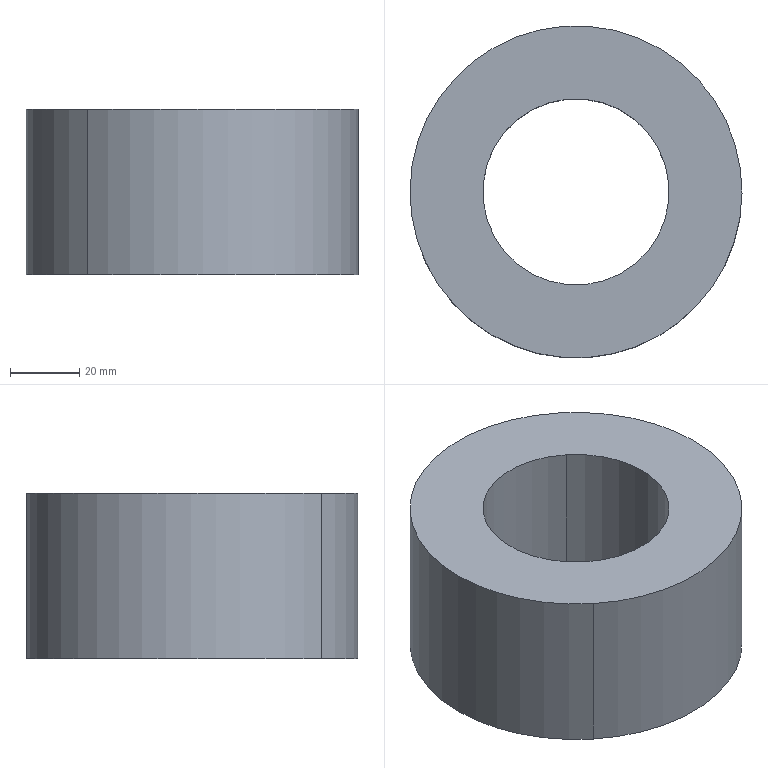Component | SolidWorks | 1-1 | 1 solid | 6 faces | box 96.06 x 96.06 x 48 mm | volume 238346 mm3 | cylinder 4 | plane 2 | commonest cylinder face diameters 53.9 x2 96.06 x2
STEP:
#1=COLOUR_RGB('',0.7922,0.8196,0.9333);
#2=FILL_AREA_STYLE_COLOUR('',#1);
#3=FILL_AREA_STYLE('',(#2));
#4=SURFACE_STYLE_FILL_AREA(#3);
#5=SURFACE_SIDE_STYLE('',(#4));
#6=SURFACE_STYLE_USAGE(.BOTH.,#5);
#7=PRESENTATION_STYLE_ASSIGNMENT((#6));
#8=CARTESIAN_POINT('',(0.6676,0.8247,-1.89));
#9=VERTEX_POINT('',#8);
#10=CARTESIAN_POINT('',(0.6676,0.8247,-3.78));
#11=VERTEX_POINT('',#10);
#12=CARTESIAN_POINT('',(0.6676,0.8247,-1.89));
#13=DIRECTION('',(0.,0.,-1.));
#14=VECTOR('',#13,39.37);
#15=LINE('',#12,#14);
#16=EDGE_CURVE('',#9,#11,#15,.T.);
#17=ORIENTED_EDGE('',*,*,#16,.F.);
#18=CARTESIAN_POINT('',(-0.6676,-0.8247,-1.89));
#19=VERTEX_POINT('',#18);
#20=CARTESIAN_POINT('',(-0.,-0.,-1.89));
#21=DIRECTION('',(0.,0.,1.));
#22=DIRECTION('',(0.6292,0.7772,0.));
#23=AXIS2_PLACEMENT_3D('',#20,#21,#22);
#24=CIRCLE('',#23,1.061);
#25=EDGE_CURVE('',#9,#19,#24,.T.);
#26=ORIENTED_EDGE('',*,*,#25,.T.);
#27=CARTESIAN_POINT('',(-0.6676,-0.8247,-3.78));
#28=VERTEX_POINT('',#27);
#29=CARTESIAN_POINT('',(-0.6676,-0.8247,-1.89));
#30=DIRECTION('',(0.,0.,-1.));
#31=VECTOR('',#30,39.37);
#32=LINE('',#29,#31);
#33=EDGE_CURVE('',#19,#28,#32,.T.);
#34=ORIENTED_EDGE('',*,*,#33,.T.);
#35=CARTESIAN_POINT('',(-0.,-0.,-3.78));
#36=DIRECTION('',(0.,0.,1.));
#37=DIRECTION('',(0.6292,0.7772,0.));
#38=AXIS2_PLACEMENT_3D('',#35,#36,#37);
#39=CIRCLE('',#38,1.061);
#40=EDGE_CURVE('',#11,#28,#39,.T.);
#41=ORIENTED_EDGE('',*,*,#40,.F.);
#42=EDGE_LOOP('',(#17,#26,#34,#41));
#43=FACE_OUTER_BOUND('',#42,.T.);
#44=CARTESIAN_POINT('',(-0.,-0.,-1.89));
#45=DIRECTION('',(0.,0.,-1.));
#46=DIRECTION('',(-0.6292,-0.7772,0.));
#47=AXIS2_PLACEMENT_3D('',#44,#45,#46);
#48=CYLINDRICAL_SURFACE('',#47,1.061);
#49=ADVANCED_FACE('',(#43),#48,.F.);
#50=CARTESIAN_POINT('',(1.19,1.47,-1.89));
#51=VERTEX_POINT('',#50);
#52=CARTESIAN_POINT('',(1.19,1.47,-3.78));
#53=VERTEX_POINT('',#52);
#54=CARTESIAN_POINT('',(1.19,1.47,-1.89));
#55=DIRECTION('',(0.,0.,-1.));
#56=VECTOR('',#55,39.37);
#57=LINE('',#54,#56);
#58=EDGE_CURVE('',#51,#53,#57,.T.);
#59=ORIENTED_EDGE('',*,*,#58,.F.);
#60=CARTESIAN_POINT('',(-1.19,-1.47,-1.89));
#61=VERTEX_POINT('',#60);
#62=CARTESIAN_POINT('',(-0.,-0.,-1.89));
#63=DIRECTION('',(0.,0.,1.));
#64=DIRECTION('',(0.6292,0.7772,0.));
#65=AXIS2_PLACEMENT_3D('',#62,#63,#64);
#66=CIRCLE('',#65,1.891);
#67=EDGE_CURVE('',#61,#51,#66,.T.);
#68=ORIENTED_EDGE('',*,*,#67,.F.);
#69=CARTESIAN_POINT('',(-1.19,-1.47,-3.78));
#70=VERTEX_POINT('',#69);
#71=CARTESIAN_POINT('',(-1.19,-1.47,-1.89));
#72=DIRECTION('',(0.,0.,-1.));
#73=VECTOR('',#72,39.37);
#74=LINE('',#71,#73);
#75=EDGE_CURVE('',#61,#70,#74,.T.);
#76=ORIENTED_EDGE('',*,*,#75,.T.);
#77=CARTESIAN_POINT('',(-0.,-0.,-3.78));
#78=DIRECTION('',(0.,0.,1.));
#79=DIRECTION('',(0.6292,0.7772,0.));
#80=AXIS2_PLACEMENT_3D('',#77,#78,#79);
#81=CIRCLE('',#80,1.891);
#82=EDGE_CURVE('',#70,#53,#81,.T.);
#83=ORIENTED_EDGE('',*,*,#82,.T.);
#84=EDGE_LOOP('',(#59,#68,#76,#83));
#85=FACE_OUTER_BOUND('',#84,.T.);
#86=CARTESIAN_POINT('',(-0.,-0.,-1.89));
#87=DIRECTION('',(0.,0.,-1.));
#88=DIRECTION('',(-0.6292,-0.7772,0.));
#89=AXIS2_PLACEMENT_3D('',#86,#87,#88);
#90=CYLINDRICAL_SURFACE('',#89,1.891);
#91=ADVANCED_FACE('',(#85),#90,.T.);
#92=CARTESIAN_POINT('',(-0.,-0.,-3.78));
#93=DIRECTION('',(0.,0.,1.));
#94=DIRECTION('',(0.6292,0.7772,0.));
#95=AXIS2_PLACEMENT_3D('',#92,#93,#94);
#96=CIRCLE('',#95,1.061);
#97=EDGE_CURVE('',#28,#11,#96,.T.);
#98=ORIENTED_EDGE('',*,*,#97,.T.);
#99=ORIENTED_EDGE('',*,*,#40,.T.);
#100=EDGE_LOOP('',(#98,#99));
#101=FACE_BOUND('',#100,.T.);
#102=ORIENTED_EDGE('',*,*,#82,.F.);
#103=CARTESIAN_POINT('',(-0.,-0.,-3.78));
#104=DIRECTION('',(0.,0.,1.));
#105=DIRECTION('',(0.6292,0.7772,0.));
#106=AXIS2_PLACEMENT_3D('',#103,#104,#105);
#107=CIRCLE('',#106,1.891);
#108=EDGE_CURVE('',#53,#70,#107,.T.);
#109=ORIENTED_EDGE('',*,*,#108,.F.);
#110=EDGE_LOOP('',(#102,#109));
#111=FACE_OUTER_BOUND('',#110,.T.);
#112=CARTESIAN_POINT('',(-0.,-0.,-3.78));
#113=DIRECTION('',(0.,0.,1.));
#114=DIRECTION('',(0.6292,0.7772,0.));
#115=AXIS2_PLACEMENT_3D('',#112,#113,#114);
#116=PLANE('',#115);
#117=ADVANCED_FACE('',(#101,#111),#116,.F.);
#118=CARTESIAN_POINT('',(-0.,-0.,-1.89));
#119=DIRECTION('',(0.,0.,1.));
#120=DIRECTION('',(0.6292,0.7772,0.));
#121=AXIS2_PLACEMENT_3D('',#118,#119,#120);
#122=CIRCLE('',#121,1.061);
#123=EDGE_CURVE('',#19,#9,#122,.T.);
#124=ORIENTED_EDGE('',*,*,#123,.F.);
#125=ORIENTED_EDGE('',*,*,#25,.F.);
#126=EDGE_LOOP('',(#124,#125));
#127=FACE_BOUND('',#126,.T.);
#128=ORIENTED_EDGE('',*,*,#67,.T.);
#129=CARTESIAN_POINT('',(-0.,-0.,-1.89));
#130=DIRECTION('',(0.,0.,1.));
#131=DIRECTION('',(0.6292,0.7772,0.));
#132=AXIS2_PLACEMENT_3D('',#129,#130,#131);
#133=CIRCLE('',#132,1.891);
#134=EDGE_CURVE('',#51,#61,#133,.T.);
#135=ORIENTED_EDGE('',*,*,#134,.T.);
#136=EDGE_LOOP('',(#128,#135));
#137=FACE_OUTER_BOUND('',#136,.T.);
#138=CARTESIAN_POINT('',(-0.,-0.,-1.89));
#139=DIRECTION('',(0.,0.,1.));
#140=DIRECTION('',(0.6292,0.7772,0.));
#141=AXIS2_PLACEMENT_3D('',#138,#139,#140);
#142=PLANE('',#141);
#143=ADVANCED_FACE('',(#127,#137),#142,.T.);
#144=ORIENTED_EDGE('',*,*,#134,.F.);
#145=ORIENTED_EDGE('',*,*,#58,.T.);
#146=ORIENTED_EDGE('',*,*,#108,.T.);
#147=ORIENTED_EDGE('',*,*,#75,.F.);
#148=EDGE_LOOP('',(#144,#145,#146,#147));
#149=FACE_OUTER_BOUND('',#148,.T.);
#150=CARTESIAN_POINT('',(-0.,-0.,-1.89));
#151=DIRECTION('',(0.,0.,-1.));
#152=DIRECTION('',(-0.6292,-0.7772,0.));
#153=AXIS2_PLACEMENT_3D('',#150,#151,#152);
#154=CYLINDRICAL_SURFACE('',#153,1.891);
#155=ADVANCED_FACE('',(#149),#154,.T.);
#156=ORIENTED_EDGE('',*,*,#123,.T.);
#157=ORIENTED_EDGE('',*,*,#16,.T.);
#158=ORIENTED_EDGE('',*,*,#97,.F.);
#159=ORIENTED_EDGE('',*,*,#33,.F.);
#160=EDGE_LOOP('',(#156,#157,#158,#159));
#161=FACE_OUTER_BOUND('',#160,.T.);
#162=CARTESIAN_POINT('',(-0.,-0.,-1.89));
#163=DIRECTION('',(0.,0.,-1.));
#164=DIRECTION('',(-0.6292,-0.7772,0.));
#165=AXIS2_PLACEMENT_3D('',#162,#163,#164);
#166=CYLINDRICAL_SURFACE('',#165,1.061);
#167=ADVANCED_FACE('',(#161),#166,.F.);
#168=CLOSED_SHELL('',(#49,#91,#117,#143,#155,#167));
#169=MANIFOLD_SOLID_BREP('',#168);
#170=STYLED_ITEM('',(#7),#169);
#171=PRESENTATION_LAYER_ASSIGNMENT('','',(#170));
#172=CARTESIAN_POINT('',(0.,0.,0.));
#173=DIRECTION('',(0.,0.,1.));
#174=DIRECTION('',(1.,0.,0.));
#175=AXIS2_PLACEMENT_3D('',#172,#173,#174);
#176=(LENGTH_UNIT()NAMED_UNIT(*)SI_UNIT($,.METRE.));
#177=LENGTH_MEASURE_WITH_UNIT(LENGTH_MEASURE(0.0254),#176);
#178=DIMENSIONAL_EXPONENTS(1.,0.,0.,0.,0.,0.,0.);
#179=(CONVERSION_BASED_UNIT('',#177)LENGTH_UNIT()NAMED_UNIT(#178));
#180=UNCERTAINTY_MEASURE_WITH_UNIT(LENGTH_MEASURE(0.00001),#179,'','');
#181=(NAMED_UNIT(*)PLANE_ANGLE_UNIT()SI_UNIT($,.RADIAN.));
#182=(NAMED_UNIT(*)SI_UNIT($,.STERADIAN.)SOLID_ANGLE_UNIT());
#183=(GEOMETRIC_REPRESENTATION_CONTEXT(3)GLOBAL_UNCERTAINTY_ASSIGNED_CONTEXT((#180))GLOBAL_UNIT_ASSIGNED_CONTEXT((#179,#181,#182))REPRESENTATION_CONTEXT('',''));
#184=ADVANCED_BREP_SHAPE_REPRESENTATION('',(#169,#175),#183);
#185=(LENGTH_UNIT()NAMED_UNIT(*)SI_UNIT($,.METRE.));
#186=LENGTH_MEASURE_WITH_UNIT(LENGTH_MEASURE(0.0254),#185);
#187=DIMENSIONAL_EXPONENTS(1.,0.,0.,0.,0.,0.,0.);
#188=(CONVERSION_BASED_UNIT('',#186)LENGTH_UNIT()NAMED_UNIT(#187));
#189=UNCERTAINTY_MEASURE_WITH_UNIT(LENGTH_MEASURE(0.00001),#188,'','');
#190=(NAMED_UNIT(*)PLANE_ANGLE_UNIT()SI_UNIT($,.RADIAN.));
#191=(NAMED_UNIT(*)SI_UNIT($,.STERADIAN.)SOLID_ANGLE_UNIT());
#192=(GEOMETRIC_REPRESENTATION_CONTEXT(3)GLOBAL_UNCERTAINTY_ASSIGNED_CONTEXT((#189))GLOBAL_UNIT_ASSIGNED_CONTEXT((#188,#190,#191))REPRESENTATION_CONTEXT('',''));
#193=MECHANICAL_DESIGN_GEOMETRIC_PRESENTATION_REPRESENTATION('',(#170),#192);